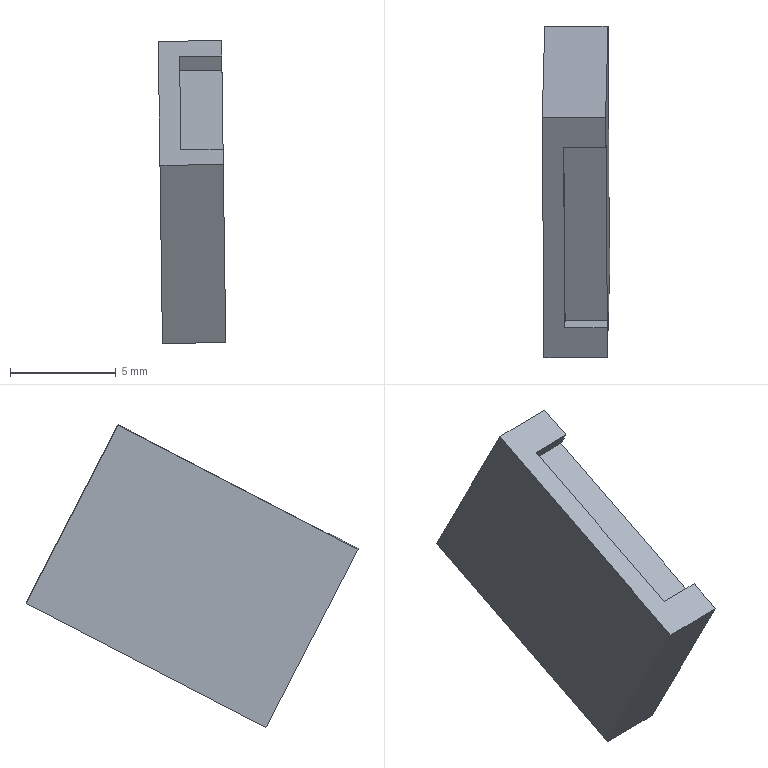Component | SolidWorks | 2018SOLIDWORKS1400000014-2 | 1 solid | 14 faces | box 3.2 x 15.73 x 14.36 mm | volume 335 mm3 | plane 14 | material White High Temperature Silicone
build123d program:
from build123d import *

# Parameters (mm, degrees)
SKETCH1_W           = 12.8
SKETCH1_H           = 9.5
BOSS_EXTRUDE1_DEPTH = 3
SKETCH3_W           = 9.6
SKETCH3_H           = 2
CUT_EXTRUDE2_DEPTH  = 0.75
SKETCH5_W           = 10
SKETCH5_H           = 1.5
CUT_EXTRUDE3_DEPTH  = 2


with BuildPart() as part:
    # Sketch1 → Boss-Extrude1 (new body)
    with BuildSketch(Plane.XY):
        Rectangle(SKETCH1_W, SKETCH1_H)
    extrude(amount=BOSS_EXTRUDE1_DEPTH)

    # Sketch3 → Cut-Extrude2 (cut)
    with BuildSketch(Plane(origin=(0, 4.75, 0), x_dir=(1, 0, 0), z_dir=(0, 1, 0))):
        with Locations((0, -2)):
            Rectangle(SKETCH3_W, SKETCH3_H)
    extrude(amount=-CUT_EXTRUDE2_DEPTH, mode=Mode.SUBTRACT)

    # Sketch5 → Cut-Extrude3 (cut)
    with BuildSketch(Plane.XY.offset(3)):
        with Locations((0, -4.75)):
            Rectangle(SKETCH5_W, SKETCH5_H)
    extrude(amount=-CUT_EXTRUDE3_DEPTH, mode=Mode.SUBTRACT)


solid = part.part

# Placed as in the assembly
solid = solid.moved(Location((101.151, -106.448, 192.228), (0, 89.207, 117.323)))